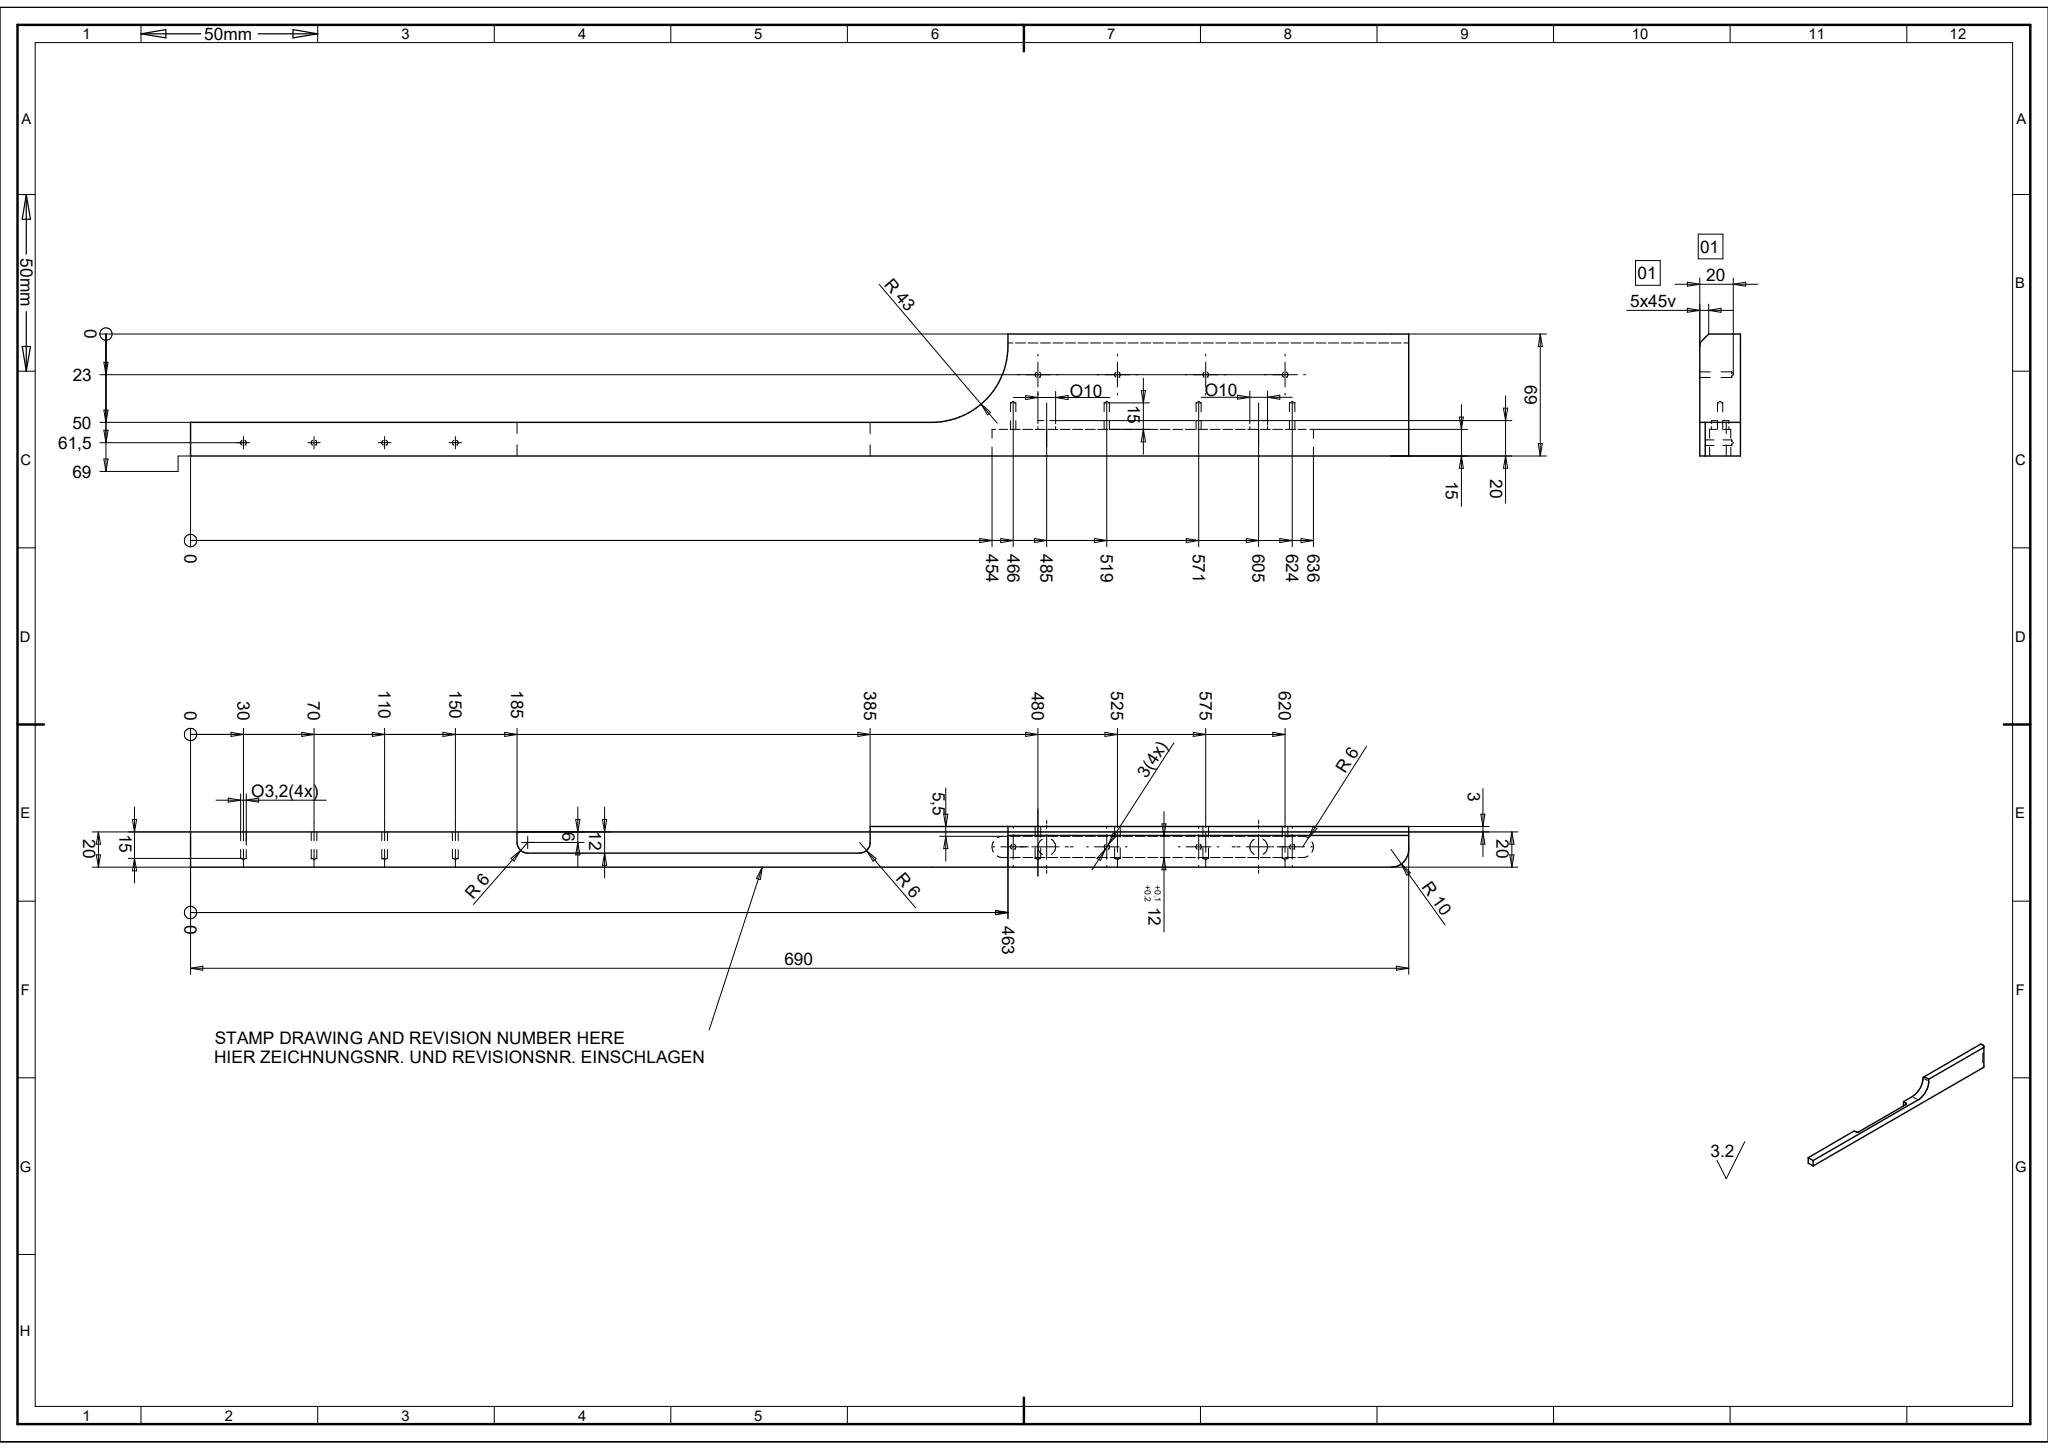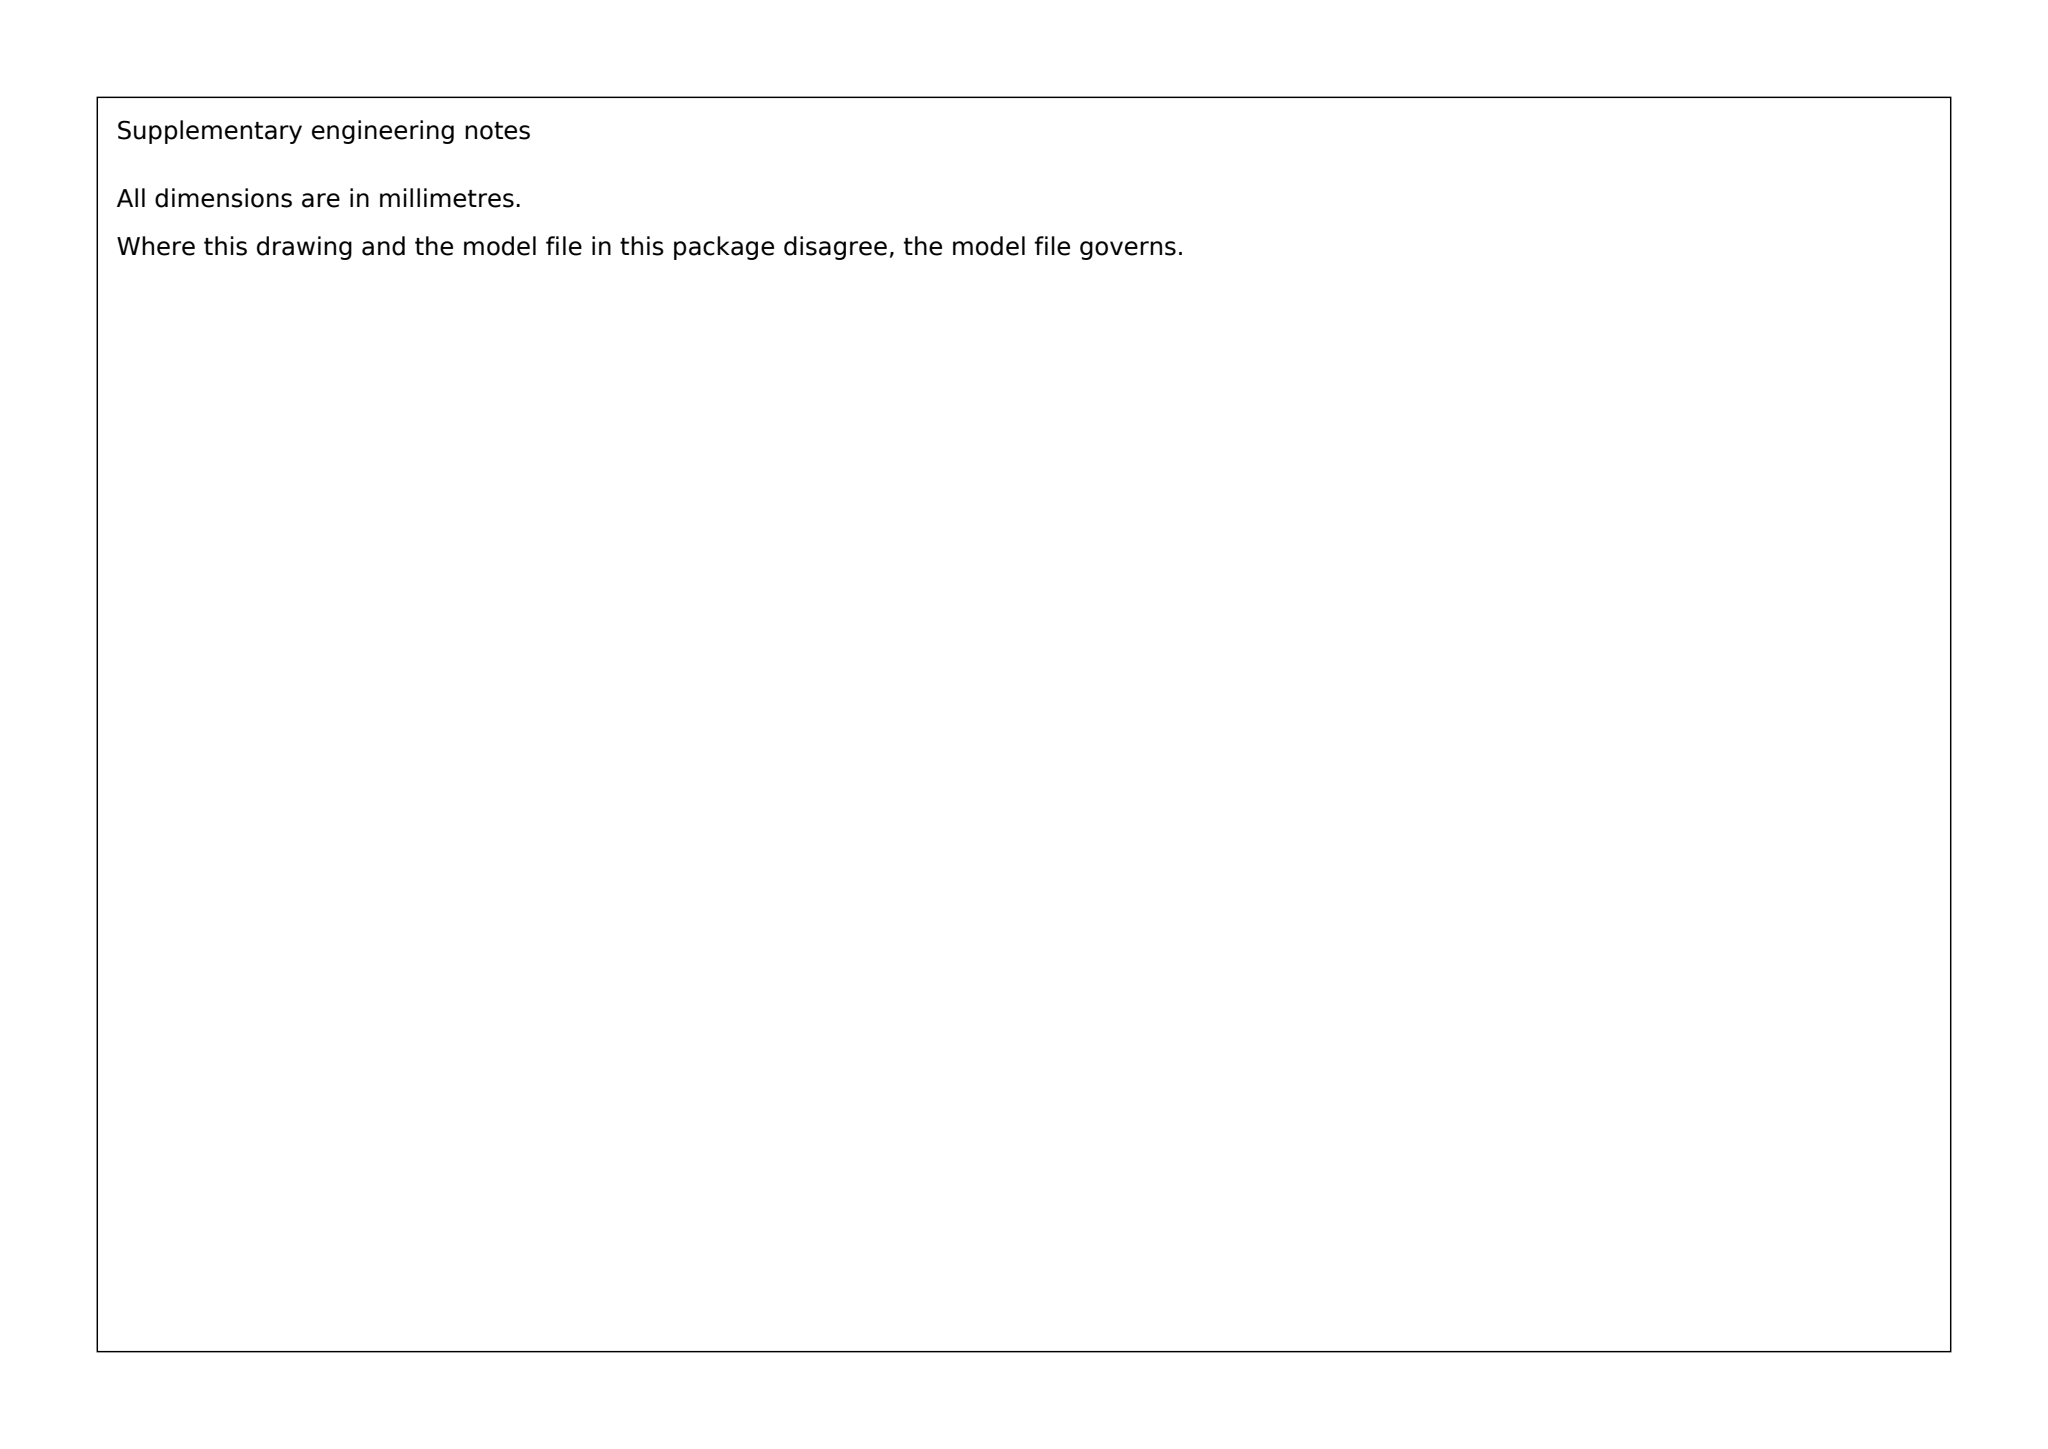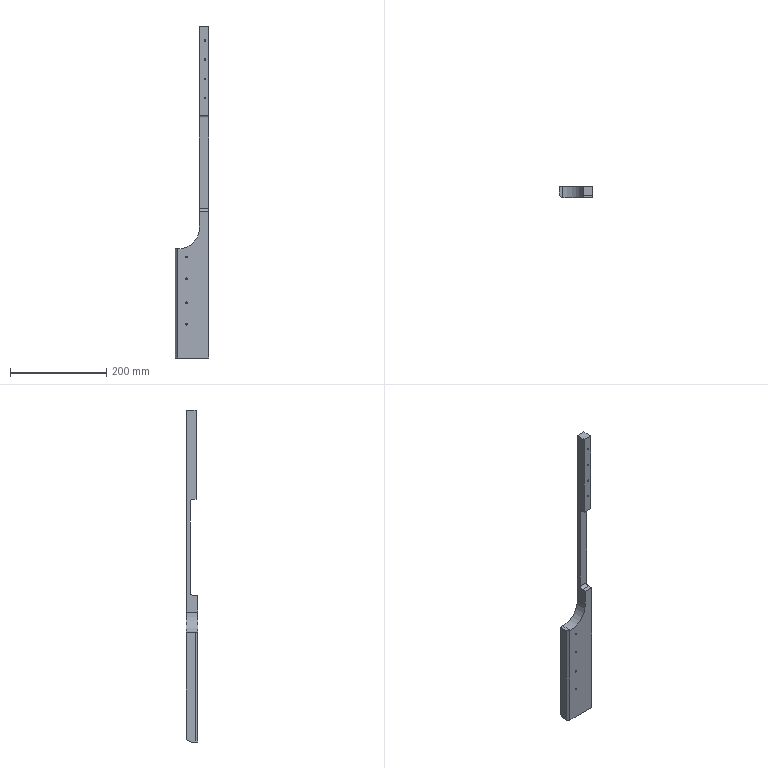Part | SolidWorks | mm | 1 solid | 77 faces | box 69 x 23 x 690 mm | volume 465637 mm3 | cylinder 35 | cone 24 | plane 18 | commonest cylinder face diameters 3.2 x16 3 x8 12 x5 10 x4 86 x1 20 x1